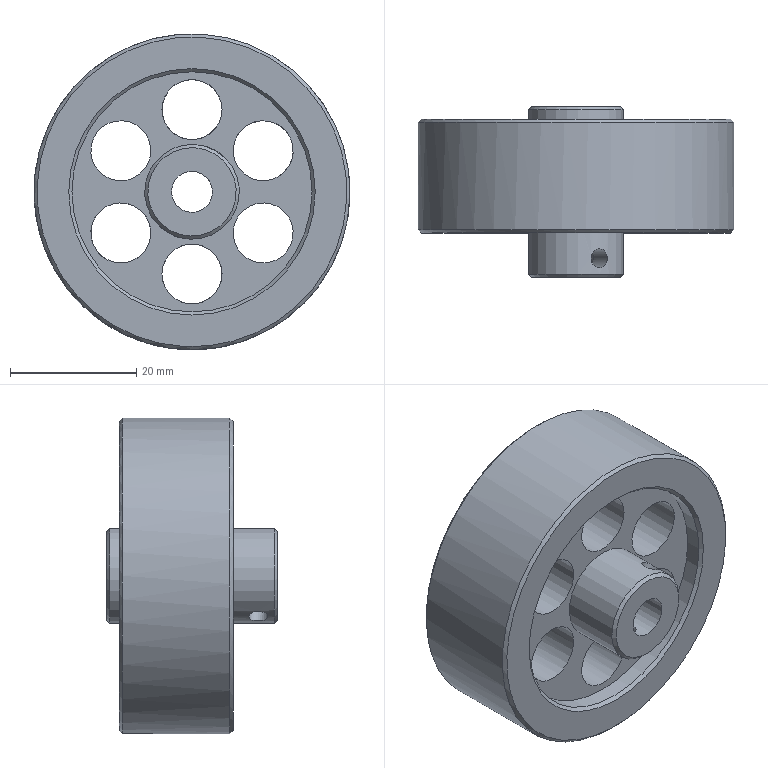Component | NX | FLYWHEEL | 1 solid | 26 faces | volume 25048 mm3 | cylinder 14 | plane 6 | cone 6 | commonest cylinder face diameters 9.5 x6 15 x2 38 x2 3 x2 6.5 x1 50 x1